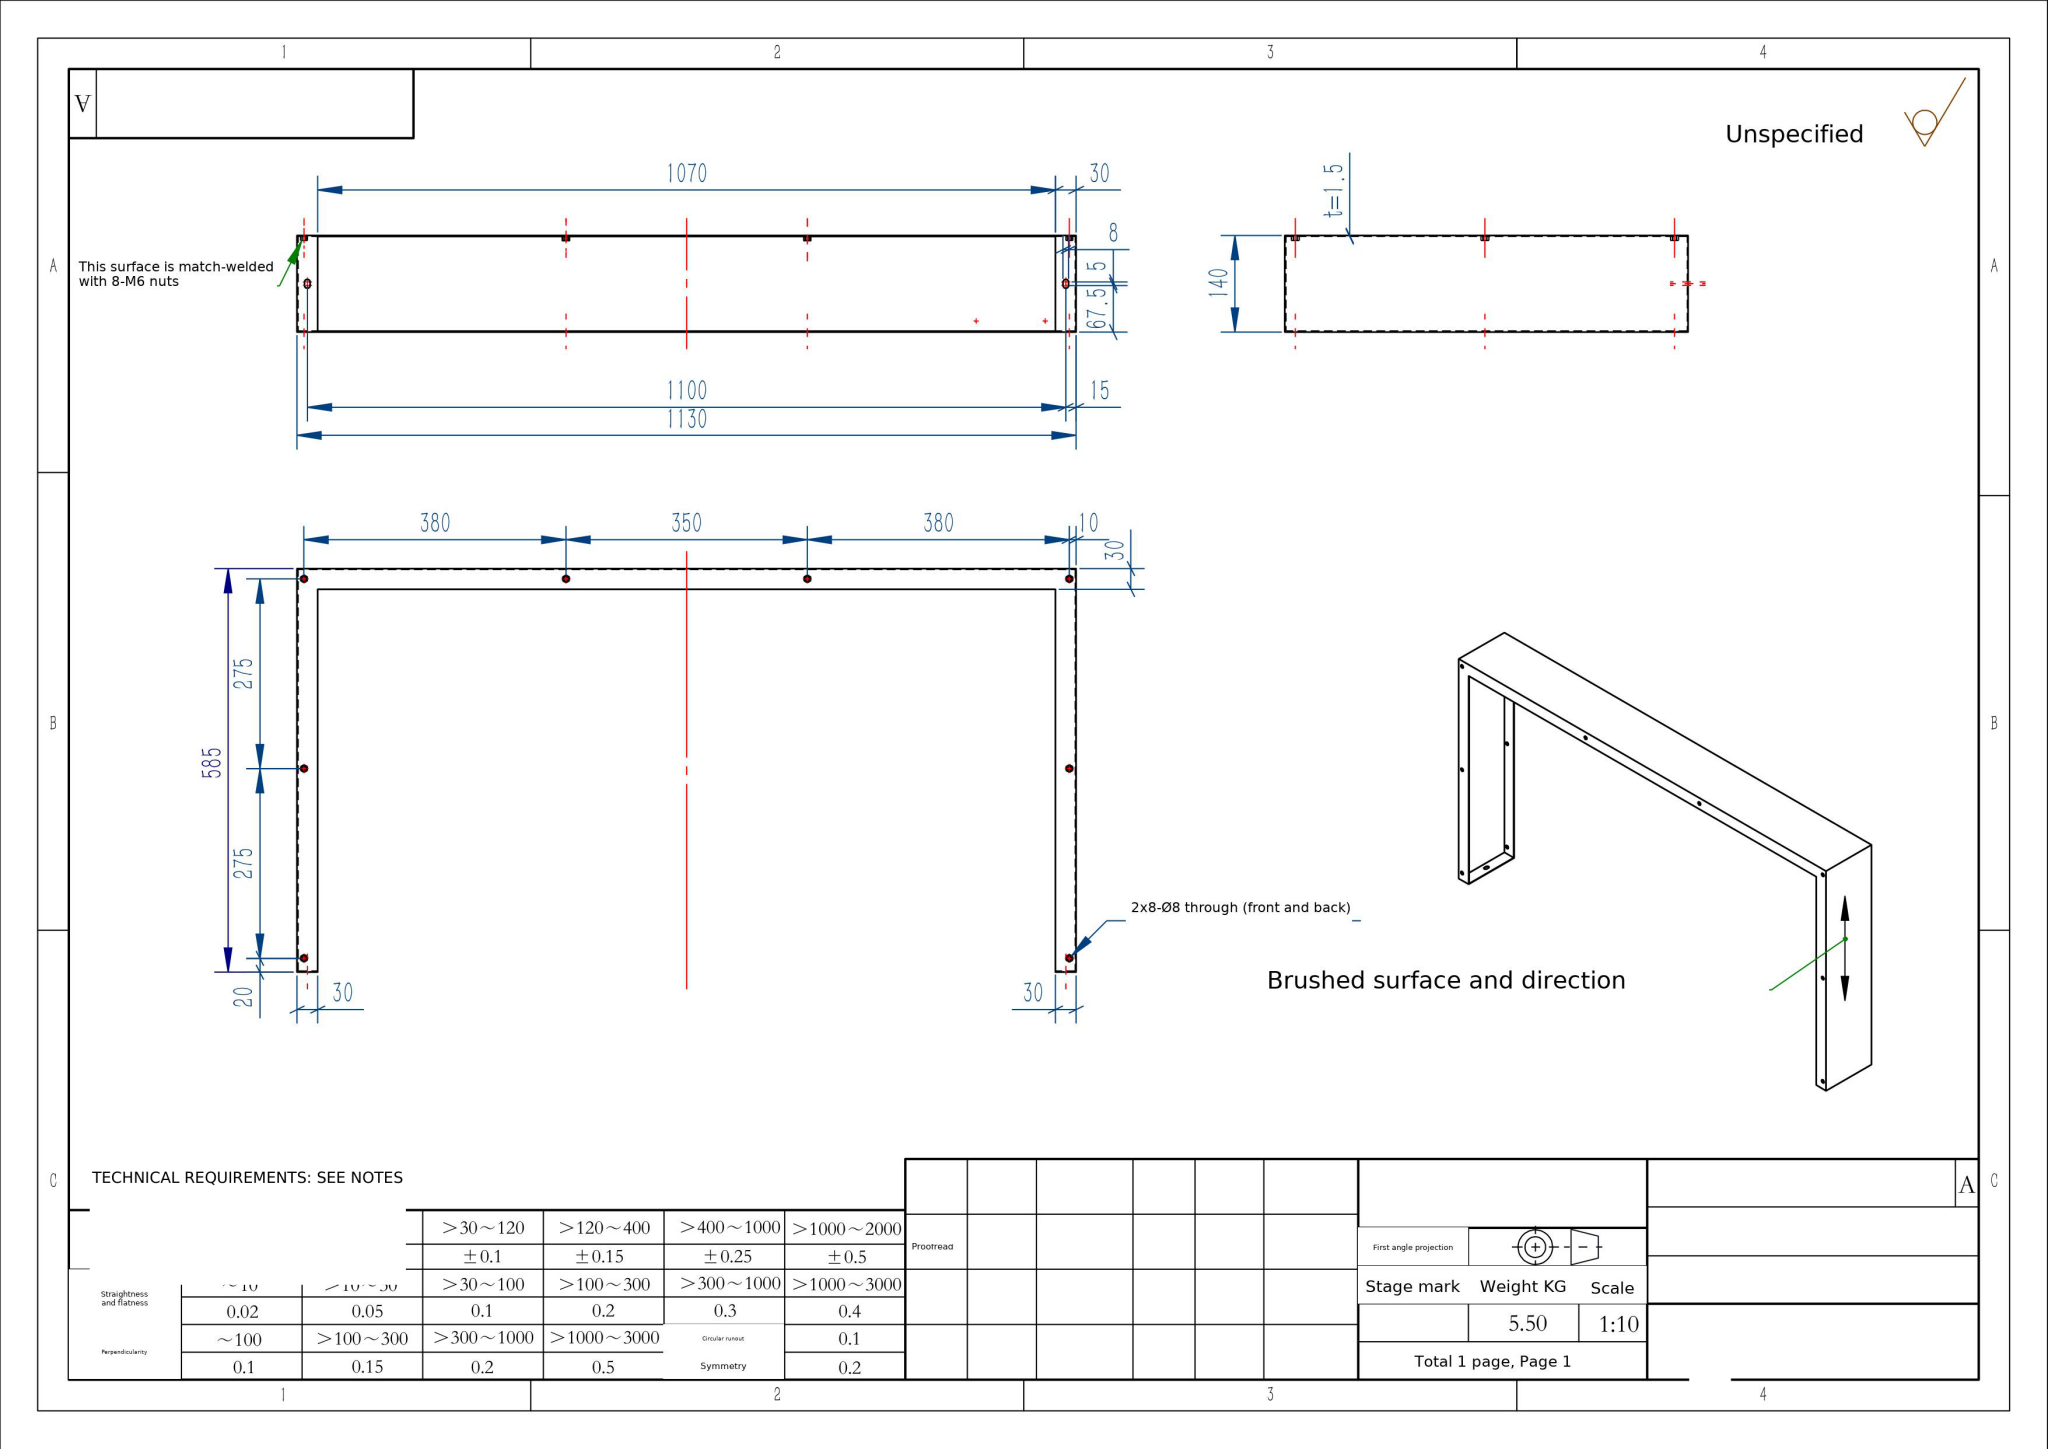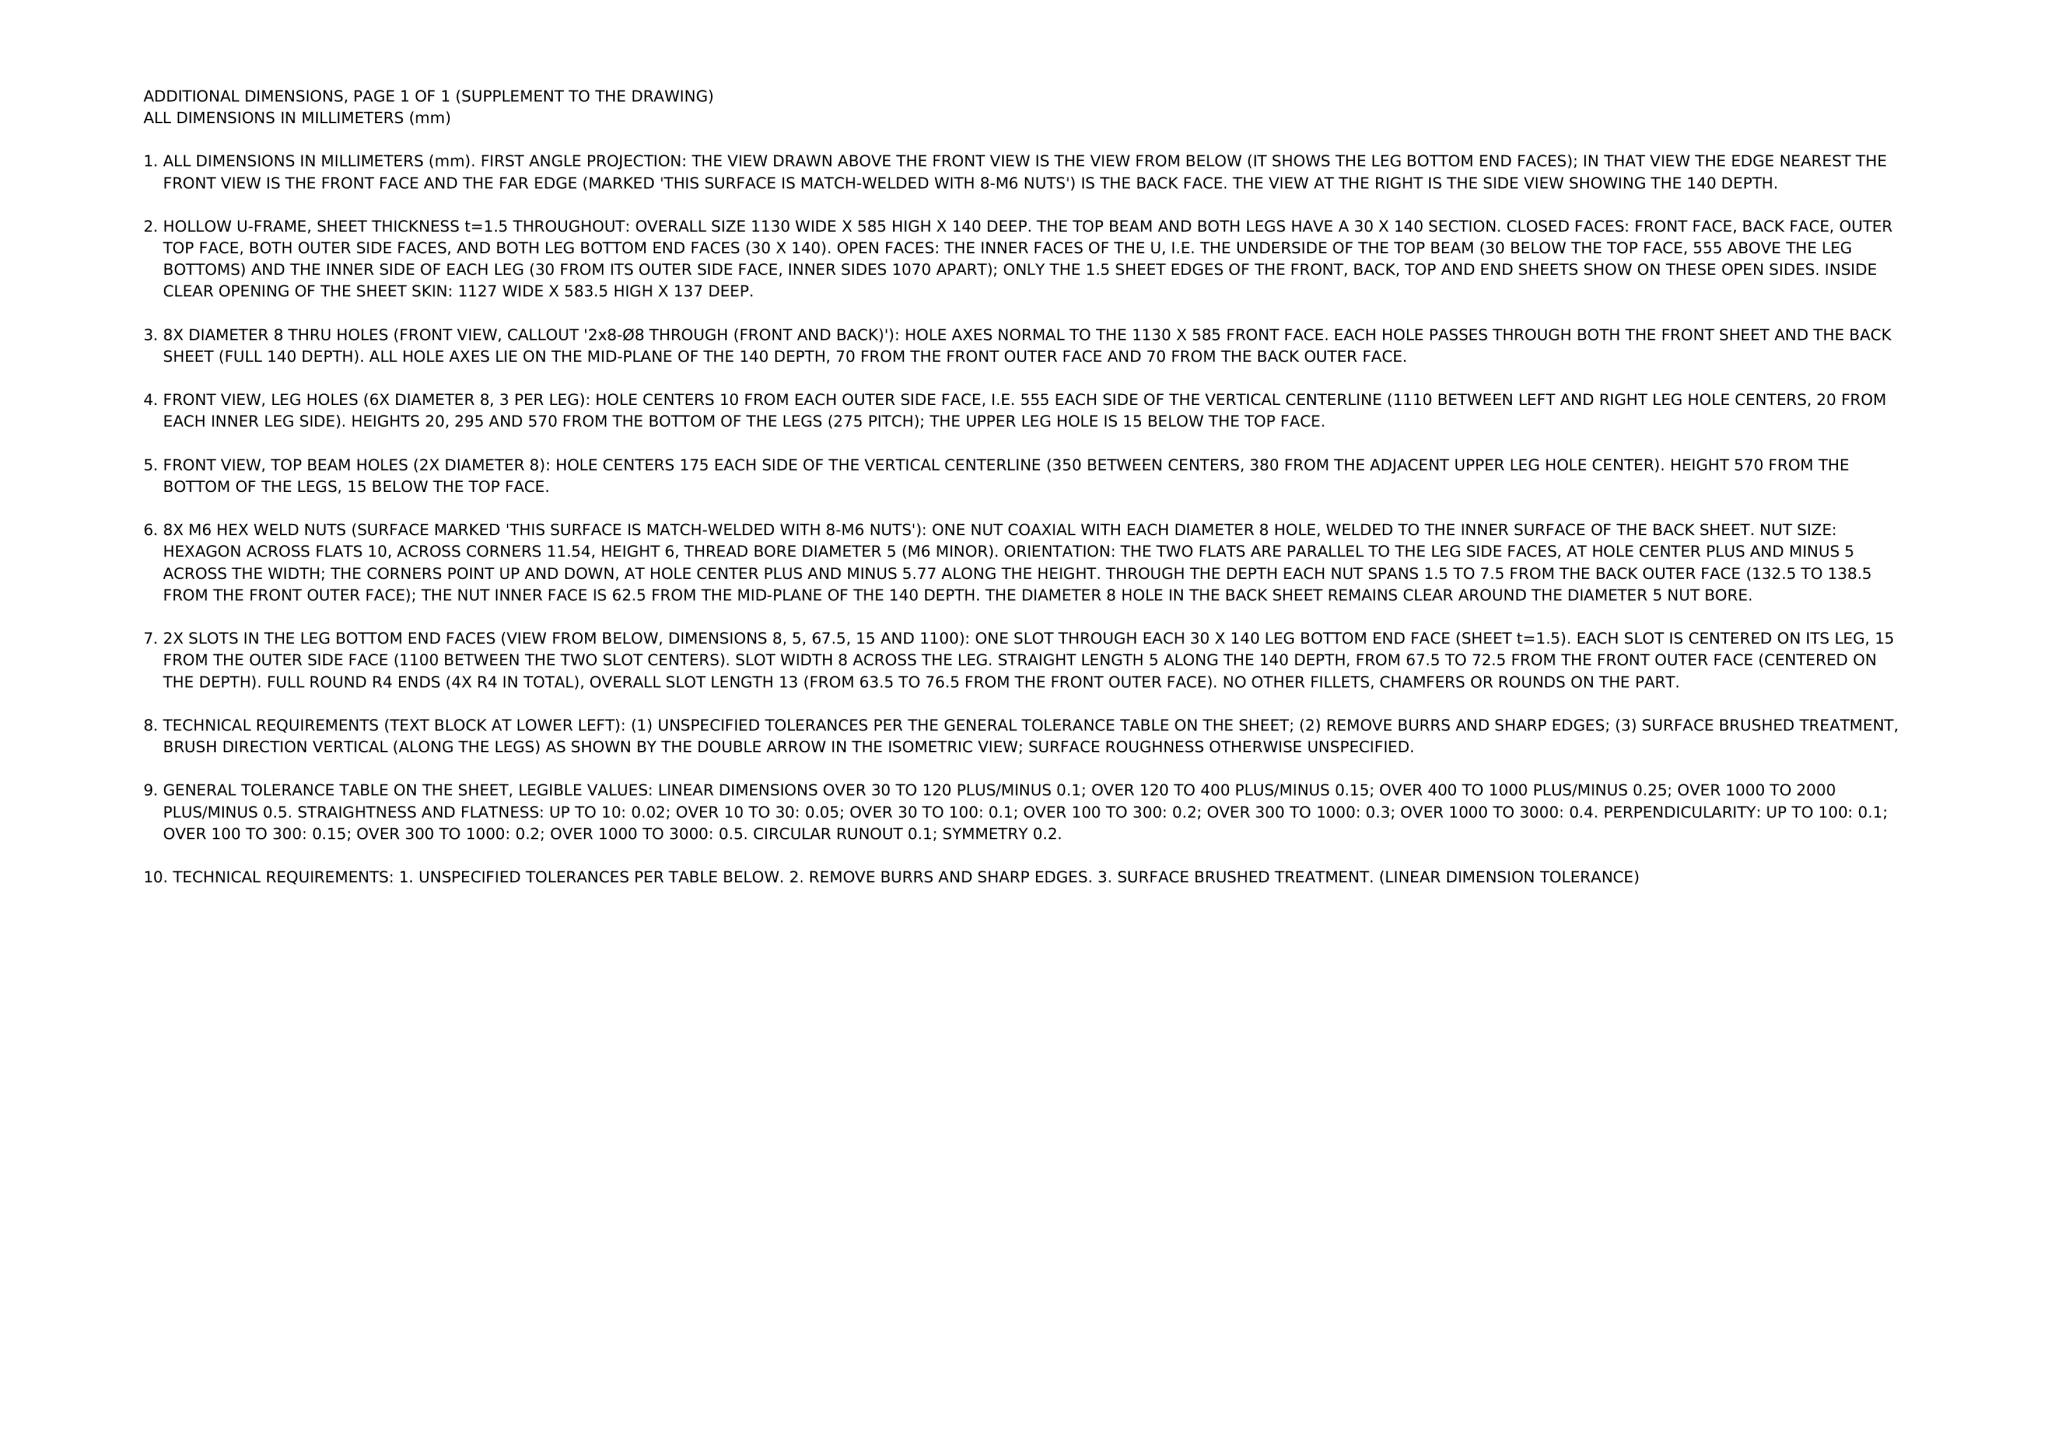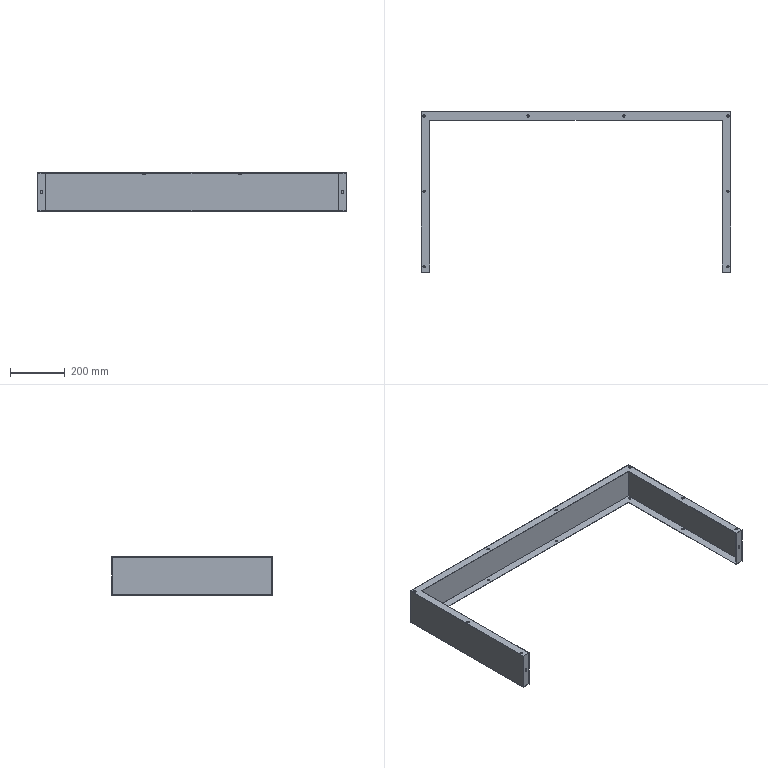Part | NX | mm | 1 solid | 140 faces | box 1130 x 585 x 140 mm | volume 687084 mm3 | plane 86 | cylinder 54 | commonest cylinder face diameters 8 x38 5 x16